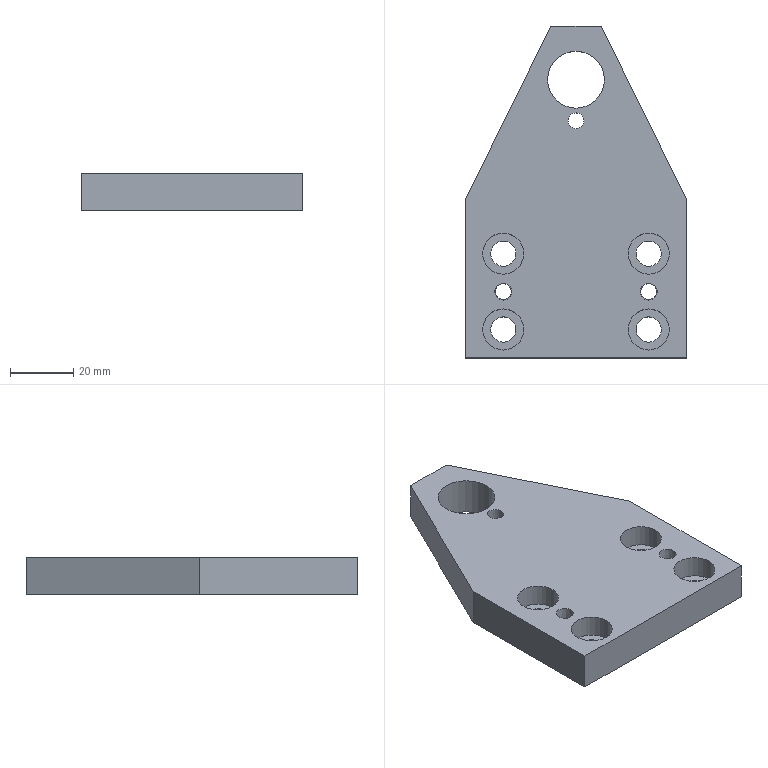Component | NX | DRILL_TEMPLATE | 1 solid | 24 faces | volume 61853 mm3 | plane 12 | cylinder 10 | cone 2 | commonest cylinder face diameters 8 x4 13 x4 5 x1 18 x1